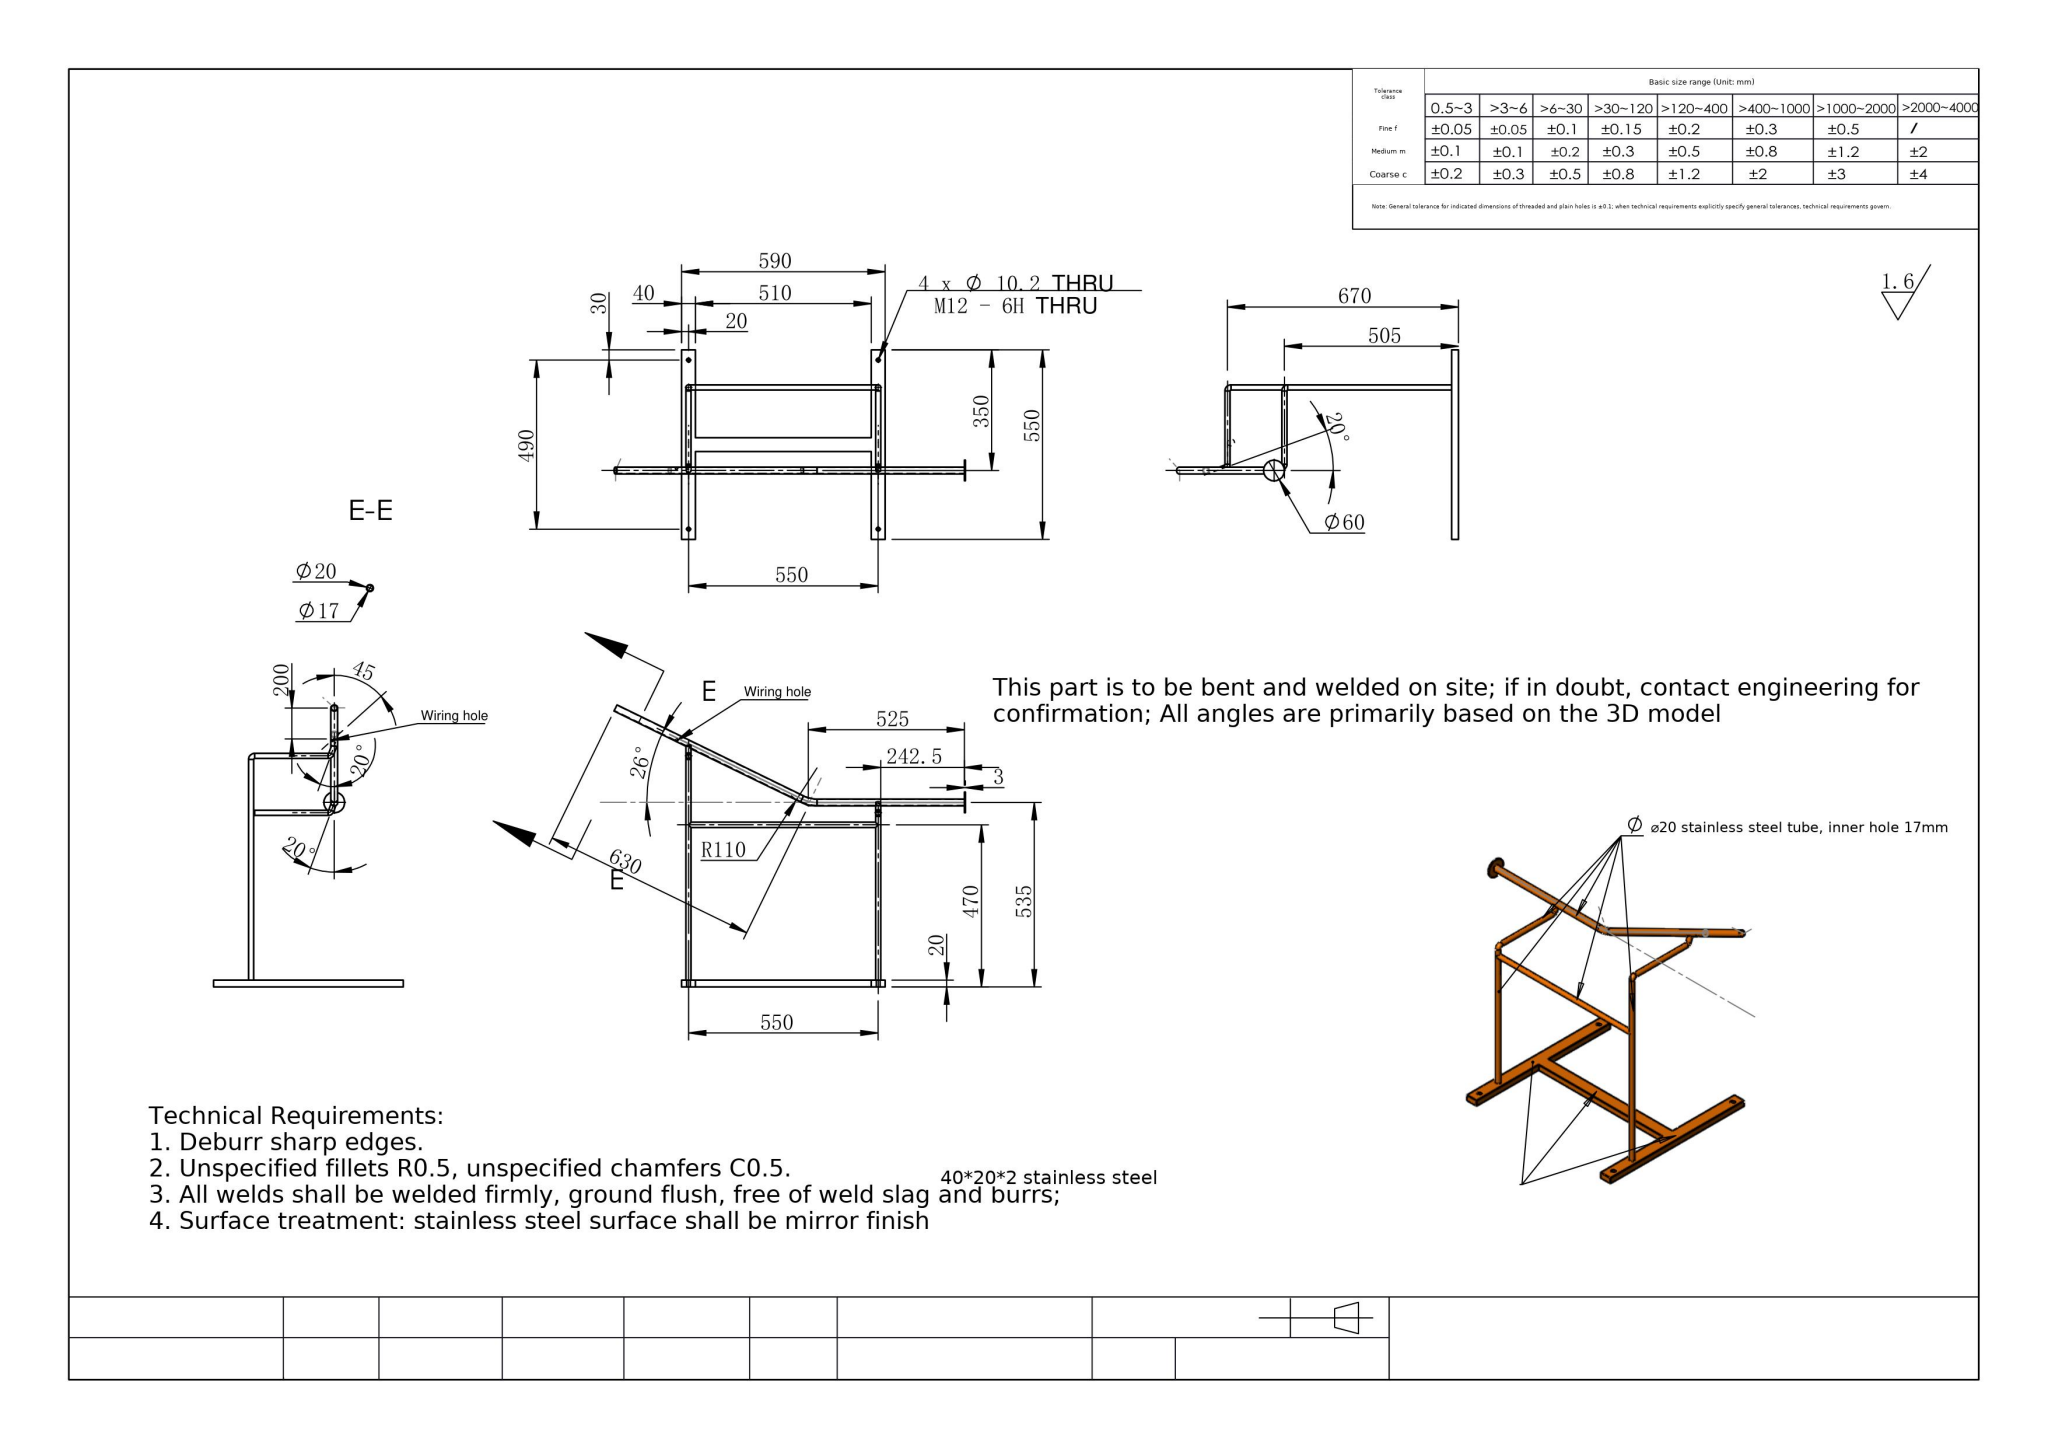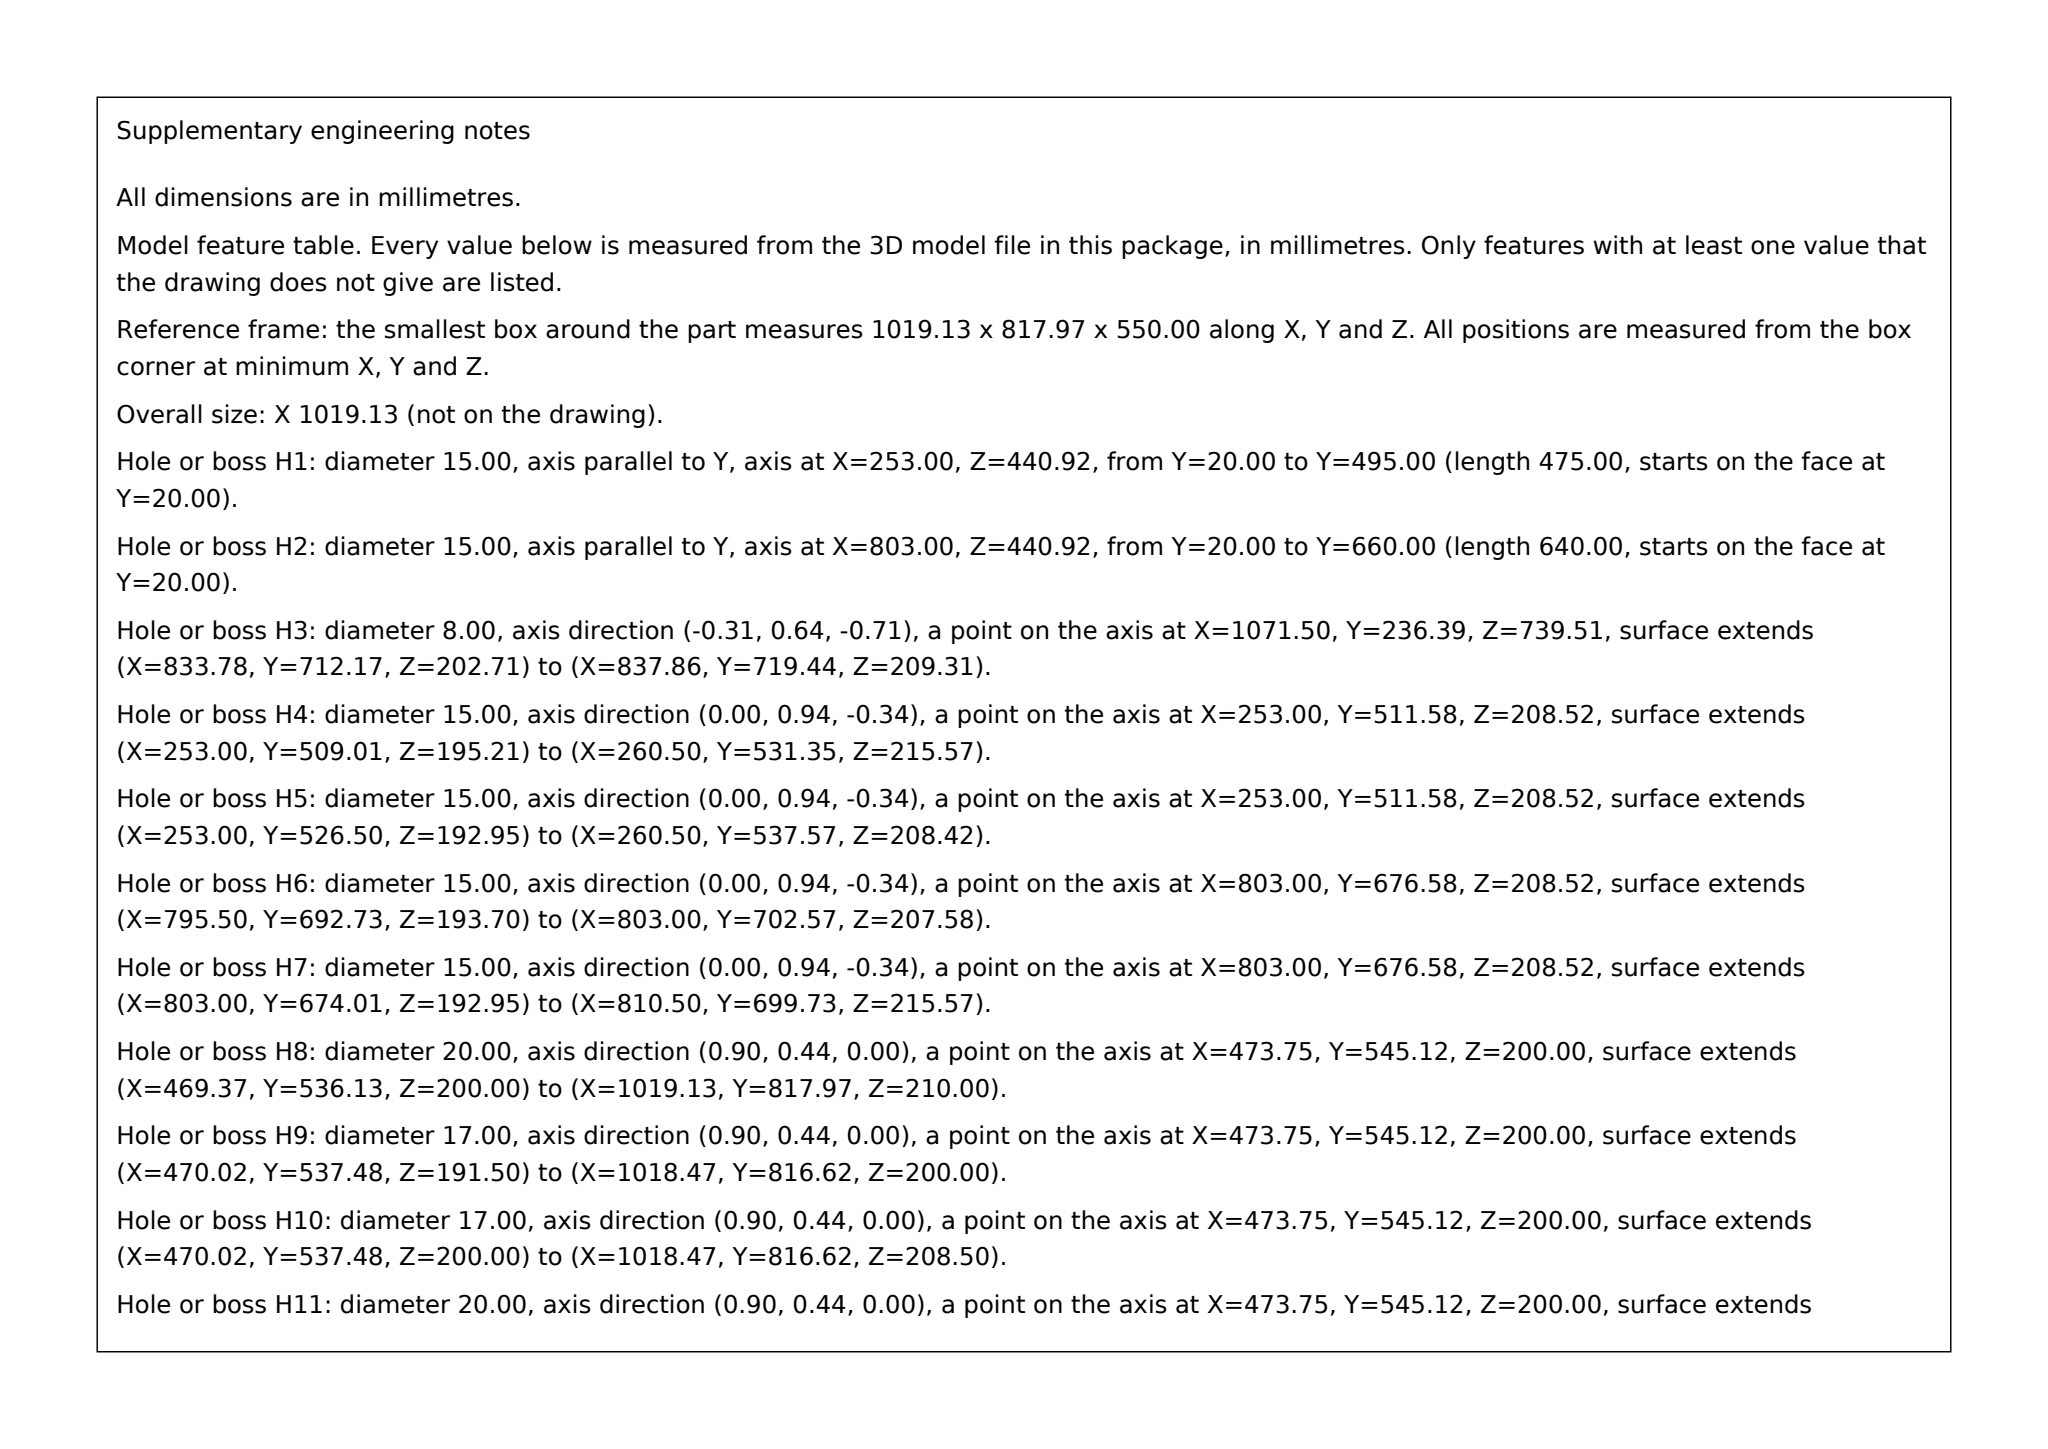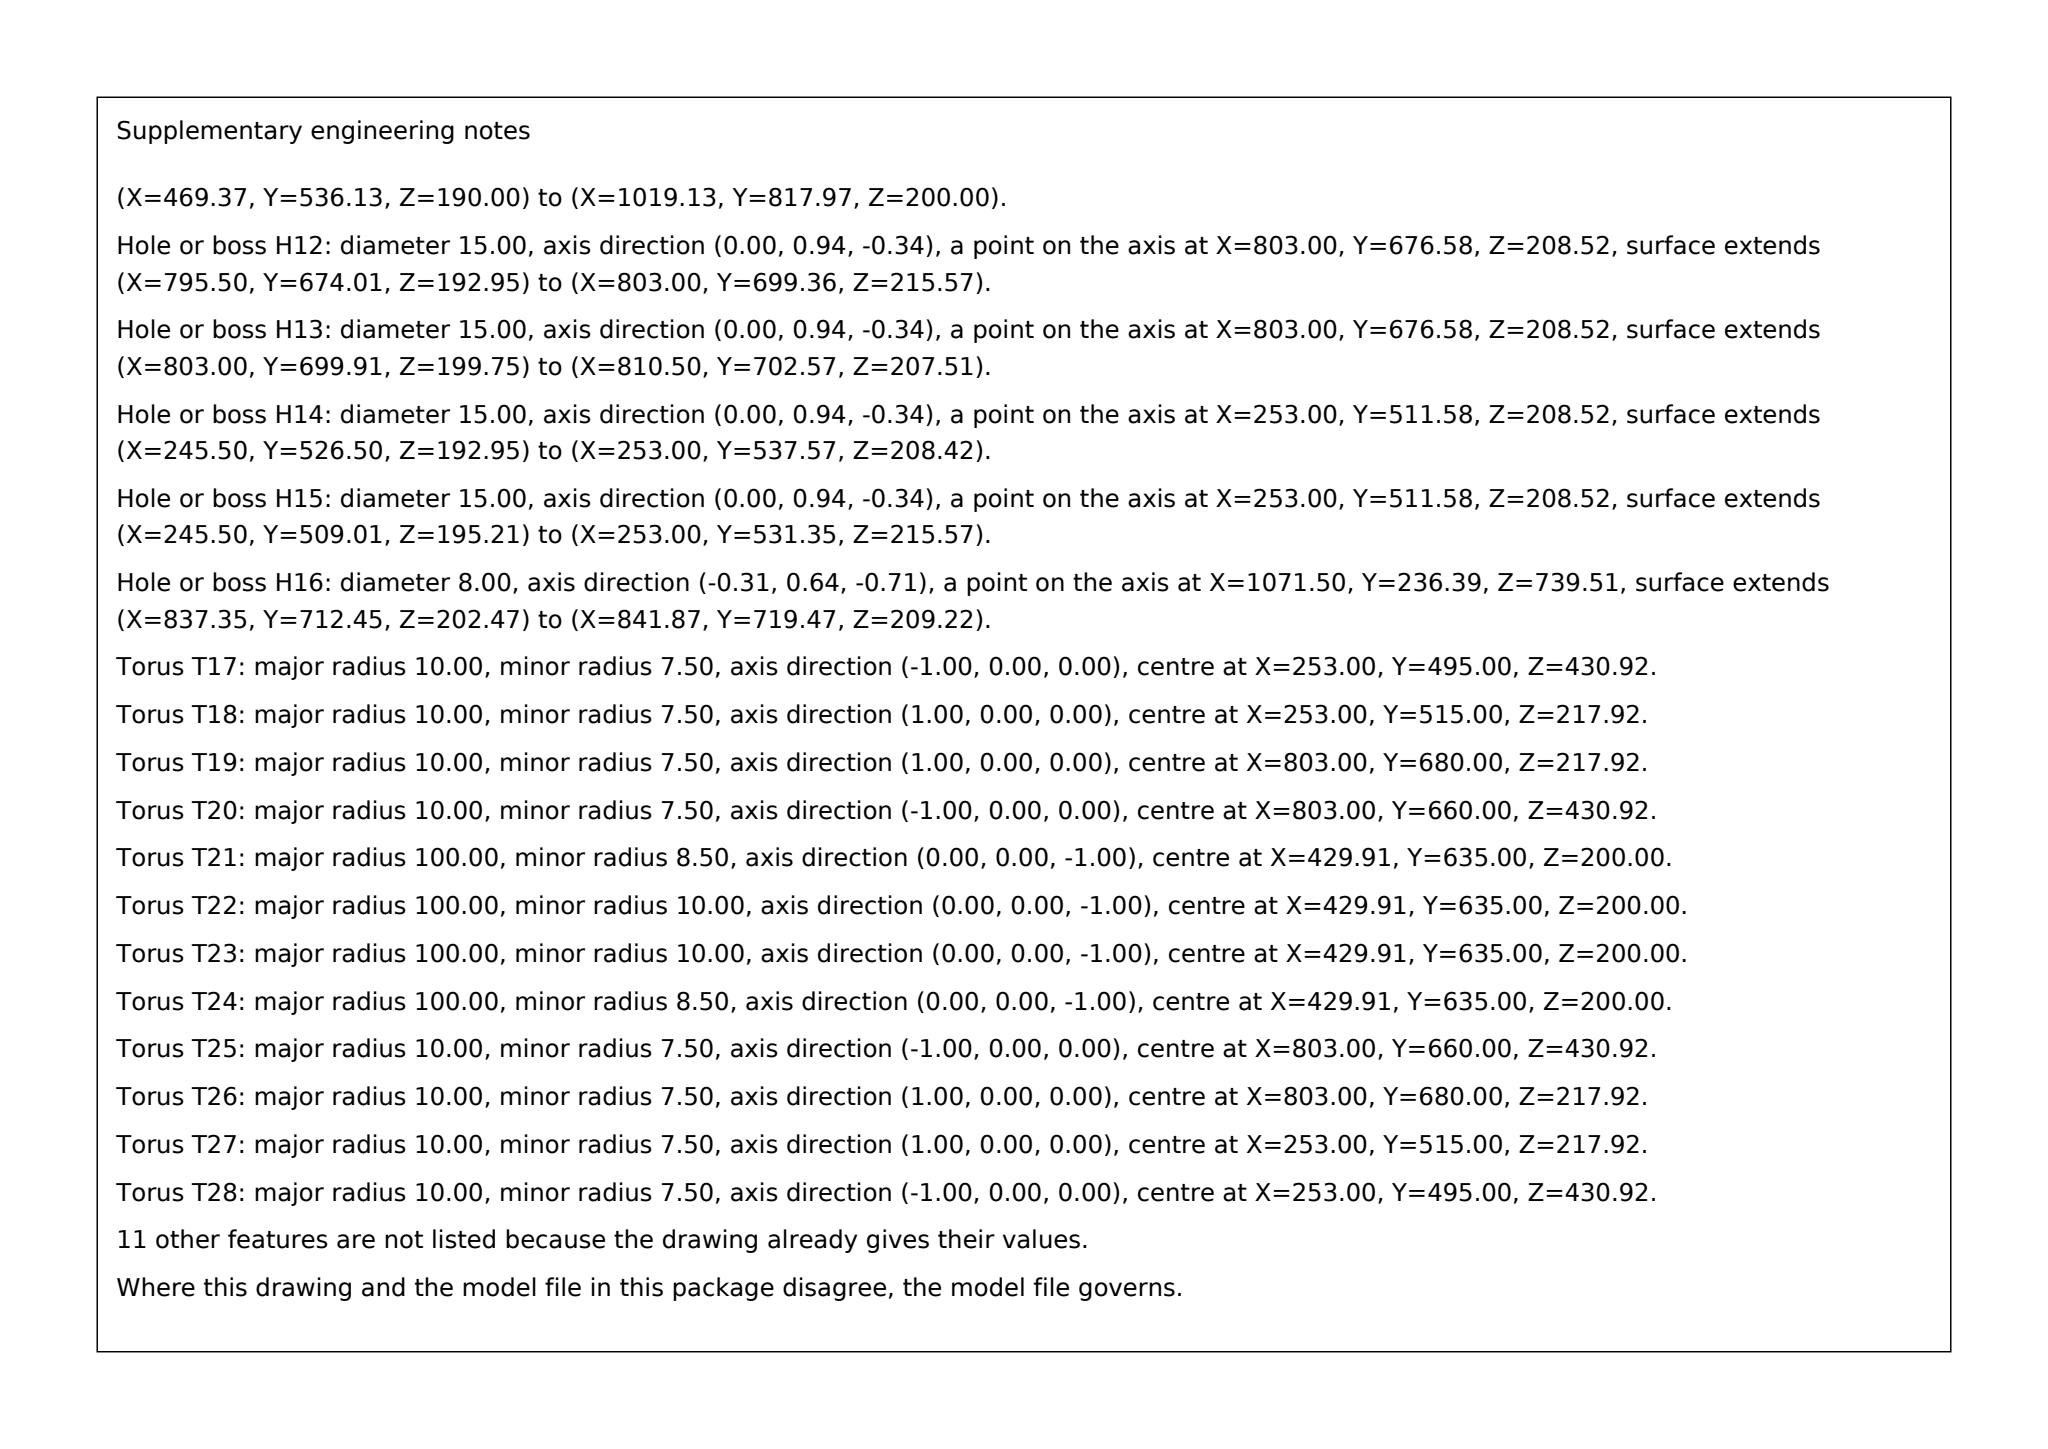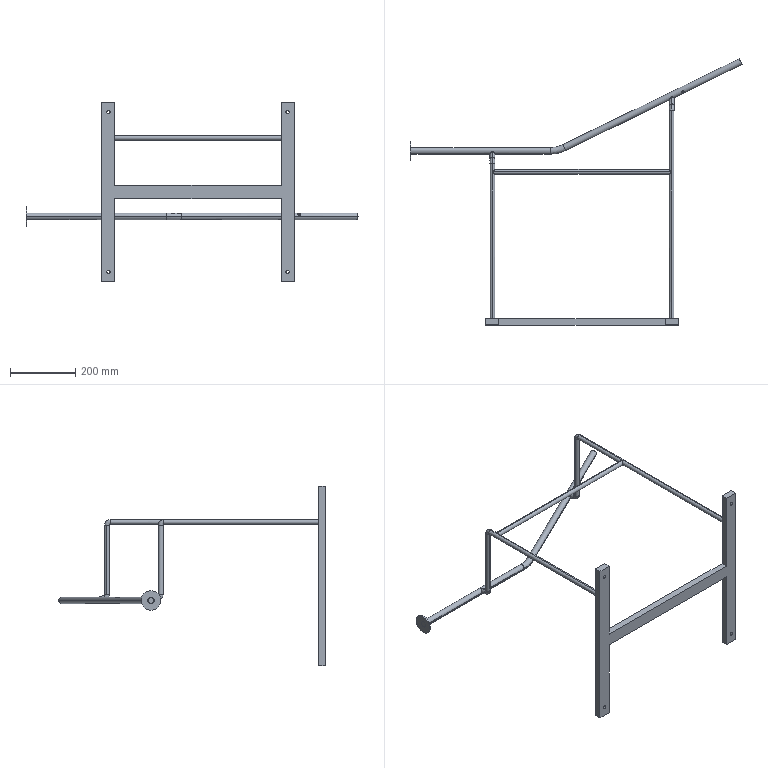Part | SolidWorks | mm | material 40*20*2 stainless steel | 1 solid | 73 faces | box 1019.13 x 817.97 x 550 mm | volume 1768854 mm3 | cylinder 40 | plane 21 | torus 12 | commonest cylinder face diameters 15 x20 10.2 x8 20 x4 17 x4 8 x2 60 x2